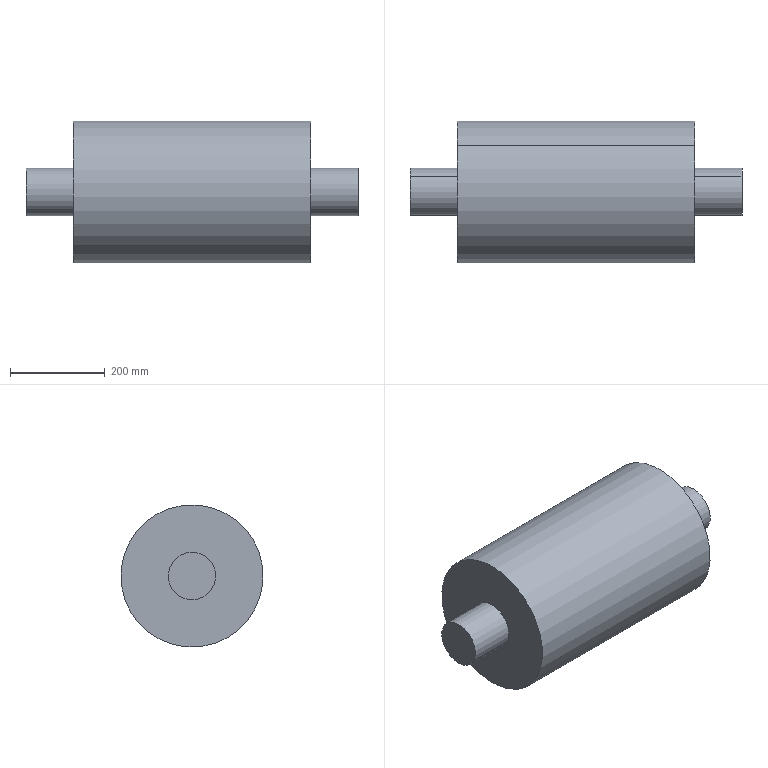Component | SolidWorks | BrushRoller-1 | 1 solid | 10 faces | box 700 x 300 x 300 mm | volume 36913714 mm3 | cylinder 6 | plane 4 | commonest cylinder face diameters 100 x4 300 x2
build123d program:
from build123d import *

# Parameters (mm, degrees)
SKETCH1_R           = 150
BOSS_EXTRUDE1_DEPTH = 500
SKETCH2_R           = 50
BOSS_EXTRUDE2_DEPTH = 100
BOSS_EXTRUDE3_START = 100
SKETCH3_R           = 50
BOSS_EXTRUDE3_DEPTH = 100


with BuildPart() as part:
    # Sketch1 → Boss-Extrude1 (new body)
    with BuildSketch(Plane.XY):
        Circle(SKETCH1_R)
    extrude(amount=BOSS_EXTRUDE1_DEPTH)

    # Sketch2 → Boss-Extrude2 (add)
    with BuildSketch(Plane.XY.offset(500)):
        Circle(SKETCH2_R)
    extrude(amount=BOSS_EXTRUDE2_DEPTH)

    # Sketch3 → Boss-Extrude3 (add)
    with BuildSketch(Plane(origin=(0, 0, 0), x_dir=(-1, 0, 0), z_dir=(0, 0, -1)).offset(BOSS_EXTRUDE3_START)):
        with Locations(Location((0, 0, 0), (0, 0, 180))):
            Circle(SKETCH3_R)
    extrude(amount=-BOSS_EXTRUDE3_DEPTH)


solid = part.part

# Placed as in the assembly
solid = solid.moved(Location((-224.371, -447.9, 85), (0, 90, 0)))
STEP:
#1=CARTESIAN_POINT('',(14.789,-18.921,1.857));
#2=VERTEX_POINT('',#1);
#3=CARTESIAN_POINT('',(14.789,-16.346,4.835));
#4=VERTEX_POINT('',#3);
#5=CARTESIAN_POINT('',(14.789,-17.634,3.346));
#6=DIRECTION('',(1.,0.,0.));
#7=DIRECTION('',(0.,-0.6541,-0.7564));
#8=AXIS2_PLACEMENT_3D('',#5,#6,#7);
#9=CIRCLE('',#8,1.969);
#10=EDGE_CURVE('',#2,#4,#9,.T.);
#11=ORIENTED_EDGE('',*,*,#10,.F.);
#12=CARTESIAN_POINT('',(10.852,-18.921,1.857));
#13=VERTEX_POINT('',#12);
#14=CARTESIAN_POINT('',(14.789,-18.921,1.857));
#15=DIRECTION('',(-1.,-0.,-0.));
#16=VECTOR('',#15,39.37);
#17=LINE('',#14,#16);
#18=EDGE_CURVE('',#2,#13,#17,.T.);
#19=ORIENTED_EDGE('',*,*,#18,.T.);
#20=CARTESIAN_POINT('',(10.852,-16.346,4.835));
#21=VERTEX_POINT('',#20);
#22=CARTESIAN_POINT('',(10.852,-17.634,3.346));
#23=DIRECTION('',(1.,0.,0.));
#24=DIRECTION('',(0.,-0.6541,-0.7564));
#25=AXIS2_PLACEMENT_3D('',#22,#23,#24);
#26=CIRCLE('',#25,1.969);
#27=EDGE_CURVE('',#13,#21,#26,.T.);
#28=ORIENTED_EDGE('',*,*,#27,.T.);
#29=CARTESIAN_POINT('',(14.789,-16.346,4.835));
#30=DIRECTION('',(-1.,-0.,-0.));
#31=VECTOR('',#30,39.37);
#32=LINE('',#29,#31);
#33=EDGE_CURVE('',#4,#21,#32,.T.);
#34=ORIENTED_EDGE('',*,*,#33,.F.);
#35=EDGE_LOOP('',(#11,#19,#28,#34));
#36=FACE_OUTER_BOUND('',#35,.T.);
#37=CARTESIAN_POINT('',(14.789,-17.634,3.346));
#38=DIRECTION('',(-1.,-0.,-0.));
#39=DIRECTION('',(0.,0.6541,0.7564));
#40=AXIS2_PLACEMENT_3D('',#37,#38,#39);
#41=CYLINDRICAL_SURFACE('',#40,1.969);
#42=ADVANCED_FACE('',(#36),#41,.T.);
#43=CARTESIAN_POINT('',(-12.77,-16.346,4.835));
#44=VERTEX_POINT('',#43);
#45=CARTESIAN_POINT('',(-12.77,-18.921,1.857));
#46=VERTEX_POINT('',#45);
#47=CARTESIAN_POINT('',(-12.77,-17.634,3.346));
#48=DIRECTION('',(-1.,-0.,-0.));
#49=DIRECTION('',(0.,0.6541,0.7564));
#50=AXIS2_PLACEMENT_3D('',#47,#48,#49);
#51=CIRCLE('',#50,1.969);
#52=EDGE_CURVE('',#44,#46,#51,.T.);
#53=ORIENTED_EDGE('',*,*,#52,.F.);
#54=CARTESIAN_POINT('',(-8.833,-16.346,4.835));
#55=VERTEX_POINT('',#54);
#56=CARTESIAN_POINT('',(-12.77,-16.346,4.835));
#57=DIRECTION('',(1.,0.,0.));
#58=VECTOR('',#57,39.37);
#59=LINE('',#56,#58);
#60=EDGE_CURVE('',#44,#55,#59,.T.);
#61=ORIENTED_EDGE('',*,*,#60,.T.);
#62=CARTESIAN_POINT('',(-8.833,-18.921,1.857));
#63=VERTEX_POINT('',#62);
#64=CARTESIAN_POINT('',(-8.833,-17.634,3.346));
#65=DIRECTION('',(-1.,-0.,-0.));
#66=DIRECTION('',(0.,0.6541,0.7564));
#67=AXIS2_PLACEMENT_3D('',#64,#65,#66);
#68=CIRCLE('',#67,1.969);
#69=EDGE_CURVE('',#55,#63,#68,.T.);
#70=ORIENTED_EDGE('',*,*,#69,.T.);
#71=CARTESIAN_POINT('',(-12.77,-18.921,1.857));
#72=DIRECTION('',(1.,0.,0.));
#73=VECTOR('',#72,39.37);
#74=LINE('',#71,#73);
#75=EDGE_CURVE('',#46,#63,#74,.T.);
#76=ORIENTED_EDGE('',*,*,#75,.F.);
#77=EDGE_LOOP('',(#53,#61,#70,#76));
#78=FACE_OUTER_BOUND('',#77,.T.);
#79=CARTESIAN_POINT('',(-12.77,-17.634,3.346));
#80=DIRECTION('',(1.,0.,0.));
#81=DIRECTION('',(0.,-0.6541,-0.7564));
#82=AXIS2_PLACEMENT_3D('',#79,#80,#81);
#83=CYLINDRICAL_SURFACE('',#82,1.969);
#84=ADVANCED_FACE('',(#78),#83,.T.);
#85=CARTESIAN_POINT('',(-8.833,-13.771,7.814));
#86=VERTEX_POINT('',#85);
#87=CARTESIAN_POINT('',(-8.833,-21.497,-1.121));
#88=VERTEX_POINT('',#87);
#89=CARTESIAN_POINT('',(-8.833,-17.634,3.346));
#90=DIRECTION('',(-1.,-0.,-0.));
#91=DIRECTION('',(-0.,0.6541,0.7564));
#92=AXIS2_PLACEMENT_3D('',#89,#90,#91);
#93=CIRCLE('',#92,5.906);
#94=EDGE_CURVE('',#86,#88,#93,.T.);
#95=ORIENTED_EDGE('',*,*,#94,.F.);
#96=CARTESIAN_POINT('',(10.852,-13.771,7.814));
#97=VERTEX_POINT('',#96);
#98=CARTESIAN_POINT('',(-8.833,-13.771,7.814));
#99=DIRECTION('',(1.,0.,0.));
#100=VECTOR('',#99,39.37);
#101=LINE('',#98,#100);
#102=EDGE_CURVE('',#86,#97,#101,.T.);
#103=ORIENTED_EDGE('',*,*,#102,.T.);
#104=CARTESIAN_POINT('',(10.852,-21.497,-1.121));
#105=VERTEX_POINT('',#104);
#106=CARTESIAN_POINT('',(10.852,-17.634,3.346));
#107=DIRECTION('',(-1.,-0.,-0.));
#108=DIRECTION('',(0.,0.6541,0.7564));
#109=AXIS2_PLACEMENT_3D('',#106,#107,#108);
#110=CIRCLE('',#109,5.906);
#111=EDGE_CURVE('',#97,#105,#110,.T.);
#112=ORIENTED_EDGE('',*,*,#111,.T.);
#113=CARTESIAN_POINT('',(-8.833,-21.497,-1.121));
#114=DIRECTION('',(1.,0.,0.));
#115=VECTOR('',#114,39.37);
#116=LINE('',#113,#115);
#117=EDGE_CURVE('',#88,#105,#116,.T.);
#118=ORIENTED_EDGE('',*,*,#117,.F.);
#119=EDGE_LOOP('',(#95,#103,#112,#118));
#120=FACE_OUTER_BOUND('',#119,.T.);
#121=CARTESIAN_POINT('',(-8.833,-17.634,3.346));
#122=DIRECTION('',(1.,0.,0.));
#123=DIRECTION('',(0.,-0.6541,-0.7564));
#124=AXIS2_PLACEMENT_3D('',#121,#122,#123);
#125=CYLINDRICAL_SURFACE('',#124,5.906);
#126=ADVANCED_FACE('',(#120),#125,.T.);
#127=ORIENTED_EDGE('',*,*,#102,.F.);
#128=CARTESIAN_POINT('',(-8.833,-17.634,3.346));
#129=DIRECTION('',(-1.,-0.,-0.));
#130=DIRECTION('',(-0.,0.6541,0.7564));
#131=AXIS2_PLACEMENT_3D('',#128,#129,#130);
#132=CIRCLE('',#131,5.906);
#133=EDGE_CURVE('',#88,#86,#132,.T.);
#134=ORIENTED_EDGE('',*,*,#133,.F.);
#135=ORIENTED_EDGE('',*,*,#117,.T.);
#136=CARTESIAN_POINT('',(10.852,-17.634,3.346));
#137=DIRECTION('',(-1.,-0.,-0.));
#138=DIRECTION('',(0.,0.6541,0.7564));
#139=AXIS2_PLACEMENT_3D('',#136,#137,#138);
#140=CIRCLE('',#139,5.906);
#141=EDGE_CURVE('',#105,#97,#140,.T.);
#142=ORIENTED_EDGE('',*,*,#141,.T.);
#143=EDGE_LOOP('',(#127,#134,#135,#142));
#144=FACE_OUTER_BOUND('',#143,.T.);
#145=CARTESIAN_POINT('',(-8.833,-17.634,3.346));
#146=DIRECTION('',(1.,0.,0.));
#147=DIRECTION('',(0.,-0.6541,-0.7564));
#148=AXIS2_PLACEMENT_3D('',#145,#146,#147);
#149=CYLINDRICAL_SURFACE('',#148,5.906);
#150=ADVANCED_FACE('',(#144),#149,.T.);
#151=CARTESIAN_POINT('',(-8.833,-17.634,3.346));
#152=DIRECTION('',(-1.,-0.,-0.));
#153=DIRECTION('',(0.,0.6541,0.7564));
#154=AXIS2_PLACEMENT_3D('',#151,#152,#153);
#155=CIRCLE('',#154,1.969);
#156=EDGE_CURVE('',#63,#55,#155,.T.);
#157=ORIENTED_EDGE('',*,*,#156,.F.);
#158=ORIENTED_EDGE('',*,*,#69,.F.);
#159=EDGE_LOOP('',(#157,#158));
#160=FACE_BOUND('',#159,.T.);
#161=ORIENTED_EDGE('',*,*,#133,.T.);
#162=ORIENTED_EDGE('',*,*,#94,.T.);
#163=EDGE_LOOP('',(#161,#162));
#164=FACE_OUTER_BOUND('',#163,.T.);
#165=CARTESIAN_POINT('',(-8.833,-17.634,3.346));
#166=DIRECTION('',(-1.,-0.,-0.));
#167=DIRECTION('',(-0.,0.6541,0.7564));
#168=AXIS2_PLACEMENT_3D('',#165,#166,#167);
#169=PLANE('',#168);
#170=ADVANCED_FACE('',(#160,#164),#169,.T.);
#171=CARTESIAN_POINT('',(10.852,-17.634,3.346));
#172=DIRECTION('',(1.,0.,0.));
#173=DIRECTION('',(0.,-0.6541,-0.7564));
#174=AXIS2_PLACEMENT_3D('',#171,#172,#173);
#175=CIRCLE('',#174,1.969);
#176=EDGE_CURVE('',#21,#13,#175,.T.);
#177=ORIENTED_EDGE('',*,*,#176,.F.);
#178=ORIENTED_EDGE('',*,*,#27,.F.);
#179=EDGE_LOOP('',(#177,#178));
#180=FACE_BOUND('',#179,.T.);
#181=ORIENTED_EDGE('',*,*,#141,.F.);
#182=ORIENTED_EDGE('',*,*,#111,.F.);
#183=EDGE_LOOP('',(#181,#182));
#184=FACE_OUTER_BOUND('',#183,.T.);
#185=CARTESIAN_POINT('',(10.852,-17.634,3.346));
#186=DIRECTION('',(-1.,-0.,-0.));
#187=DIRECTION('',(-0.,0.6541,0.7564));
#188=AXIS2_PLACEMENT_3D('',#185,#186,#187);
#189=PLANE('',#188);
#190=ADVANCED_FACE('',(#180,#184),#189,.F.);
#191=ORIENTED_EDGE('',*,*,#60,.F.);
#192=CARTESIAN_POINT('',(-12.77,-17.634,3.346));
#193=DIRECTION('',(-1.,-0.,-0.));
#194=DIRECTION('',(0.,0.6541,0.7564));
#195=AXIS2_PLACEMENT_3D('',#192,#193,#194);
#196=CIRCLE('',#195,1.969);
#197=EDGE_CURVE('',#46,#44,#196,.T.);
#198=ORIENTED_EDGE('',*,*,#197,.F.);
#199=ORIENTED_EDGE('',*,*,#75,.T.);
#200=ORIENTED_EDGE('',*,*,#156,.T.);
#201=EDGE_LOOP('',(#191,#198,#199,#200));
#202=FACE_OUTER_BOUND('',#201,.T.);
#203=CARTESIAN_POINT('',(-12.77,-17.634,3.346));
#204=DIRECTION('',(1.,0.,0.));
#205=DIRECTION('',(0.,-0.6541,-0.7564));
#206=AXIS2_PLACEMENT_3D('',#203,#204,#205);
#207=CYLINDRICAL_SURFACE('',#206,1.969);
#208=ADVANCED_FACE('',(#202),#207,.T.);
#209=ORIENTED_EDGE('',*,*,#197,.T.);
#210=ORIENTED_EDGE('',*,*,#52,.T.);
#211=EDGE_LOOP('',(#209,#210));
#212=FACE_OUTER_BOUND('',#211,.T.);
#213=CARTESIAN_POINT('',(-12.77,-17.634,3.346));
#214=DIRECTION('',(-1.,-0.,-0.));
#215=DIRECTION('',(-0.,0.6541,0.7564));
#216=AXIS2_PLACEMENT_3D('',#213,#214,#215);
#217=PLANE('',#216);
#218=ADVANCED_FACE('',(#212),#217,.T.);
#219=ORIENTED_EDGE('',*,*,#18,.F.);
#220=CARTESIAN_POINT('',(14.789,-17.634,3.346));
#221=DIRECTION('',(1.,0.,0.));
#222=DIRECTION('',(0.,-0.6541,-0.7564));
#223=AXIS2_PLACEMENT_3D('',#220,#221,#222);
#224=CIRCLE('',#223,1.969);
#225=EDGE_CURVE('',#4,#2,#224,.T.);
#226=ORIENTED_EDGE('',*,*,#225,.F.);
#227=ORIENTED_EDGE('',*,*,#33,.T.);
#228=ORIENTED_EDGE('',*,*,#176,.T.);
#229=EDGE_LOOP('',(#219,#226,#227,#228));
#230=FACE_OUTER_BOUND('',#229,.T.);
#231=CARTESIAN_POINT('',(14.789,-17.634,3.346));
#232=DIRECTION('',(-1.,-0.,-0.));
#233=DIRECTION('',(0.,0.6541,0.7564));
#234=AXIS2_PLACEMENT_3D('',#231,#232,#233);
#235=CYLINDRICAL_SURFACE('',#234,1.969);
#236=ADVANCED_FACE('',(#230),#235,.T.);
#237=ORIENTED_EDGE('',*,*,#225,.T.);
#238=ORIENTED_EDGE('',*,*,#10,.T.);
#239=EDGE_LOOP('',(#237,#238));
#240=FACE_OUTER_BOUND('',#239,.T.);
#241=CARTESIAN_POINT('',(14.789,-17.634,3.346));
#242=DIRECTION('',(1.,0.,0.));
#243=DIRECTION('',(0.,-0.6541,-0.7564));
#244=AXIS2_PLACEMENT_3D('',#241,#242,#243);
#245=PLANE('',#244);
#246=ADVANCED_FACE('',(#240),#245,.T.);
#247=CLOSED_SHELL('',(#42,#84,#126,#150,#170,#190,#208,#218,#236,#246));
#248=MANIFOLD_SOLID_BREP('',#247);
#249=CARTESIAN_POINT('',(0.,0.,0.));
#250=DIRECTION('',(0.,0.,1.));
#251=DIRECTION('',(1.,0.,0.));
#252=AXIS2_PLACEMENT_3D('',#249,#250,#251);
#253=(LENGTH_UNIT()NAMED_UNIT(*)SI_UNIT($,.METRE.));
#254=LENGTH_MEASURE_WITH_UNIT(LENGTH_MEASURE(0.0254),#253);
#255=DIMENSIONAL_EXPONENTS(1.,0.,0.,0.,0.,0.,0.);
#256=(CONVERSION_BASED_UNIT('',#254)LENGTH_UNIT()NAMED_UNIT(#255));
#257=UNCERTAINTY_MEASURE_WITH_UNIT(LENGTH_MEASURE(0.00001),#256,'','');
#258=(NAMED_UNIT(*)PLANE_ANGLE_UNIT()SI_UNIT($,.RADIAN.));
#259=(NAMED_UNIT(*)SI_UNIT($,.STERADIAN.)SOLID_ANGLE_UNIT());
#260=(GEOMETRIC_REPRESENTATION_CONTEXT(3)GLOBAL_UNCERTAINTY_ASSIGNED_CONTEXT((#257))GLOBAL_UNIT_ASSIGNED_CONTEXT((#256,#258,#259))REPRESENTATION_CONTEXT('',''));
#261=ADVANCED_BREP_SHAPE_REPRESENTATION('',(#248,#252),#260);
#262=COLOUR_RGB('',0.7922,0.8196,0.9333);
#263=FILL_AREA_STYLE_COLOUR('',#262);
#264=FILL_AREA_STYLE('',(#263));
#265=SURFACE_STYLE_FILL_AREA(#264);
#266=SURFACE_SIDE_STYLE('',(#265));
#267=SURFACE_STYLE_USAGE(.BOTH.,#266);
#268=PRESENTATION_STYLE_ASSIGNMENT((#267));
#269=STYLED_ITEM('',(#268),#248);
#270=(LENGTH_UNIT()NAMED_UNIT(*)SI_UNIT($,.METRE.));
#271=LENGTH_MEASURE_WITH_UNIT(LENGTH_MEASURE(0.0254),#270);
#272=DIMENSIONAL_EXPONENTS(1.,0.,0.,0.,0.,0.,0.);
#273=(CONVERSION_BASED_UNIT('',#271)LENGTH_UNIT()NAMED_UNIT(#272));
#274=UNCERTAINTY_MEASURE_WITH_UNIT(LENGTH_MEASURE(0.00001),#273,'','');
#275=(NAMED_UNIT(*)PLANE_ANGLE_UNIT()SI_UNIT($,.RADIAN.));
#276=(NAMED_UNIT(*)SI_UNIT($,.STERADIAN.)SOLID_ANGLE_UNIT());
#277=(GEOMETRIC_REPRESENTATION_CONTEXT(3)GLOBAL_UNCERTAINTY_ASSIGNED_CONTEXT((#274))GLOBAL_UNIT_ASSIGNED_CONTEXT((#273,#275,#276))REPRESENTATION_CONTEXT('',''));
#278=MECHANICAL_DESIGN_GEOMETRIC_PRESENTATION_REPRESENTATION('',(#269),#277);
#279=PRESENTATION_LAYER_ASSIGNMENT('','',(#269));